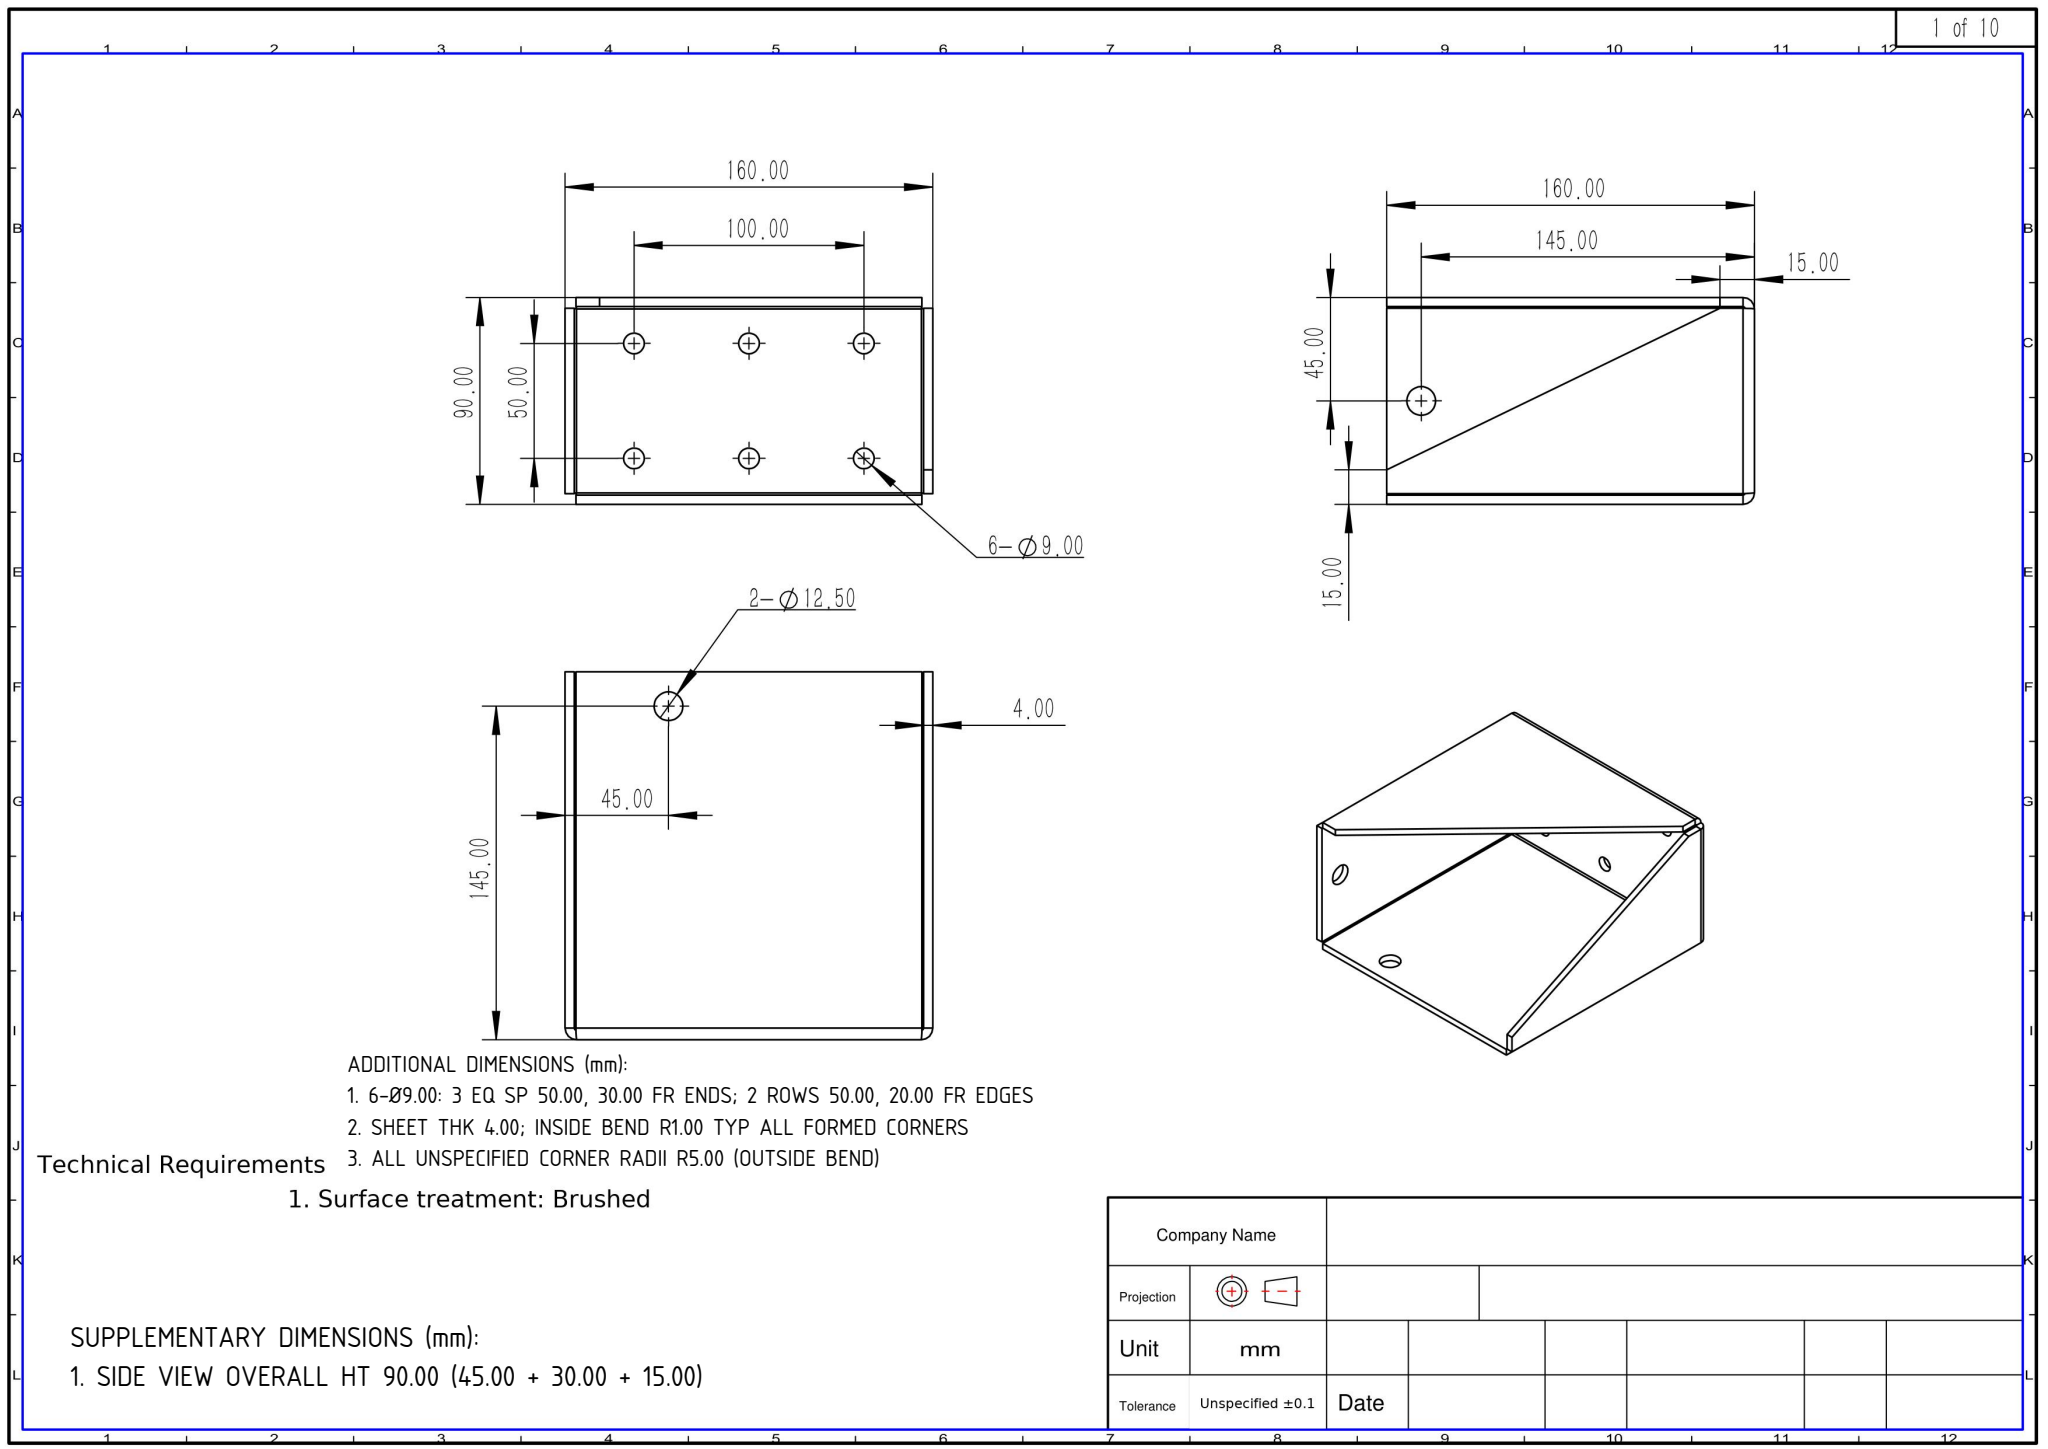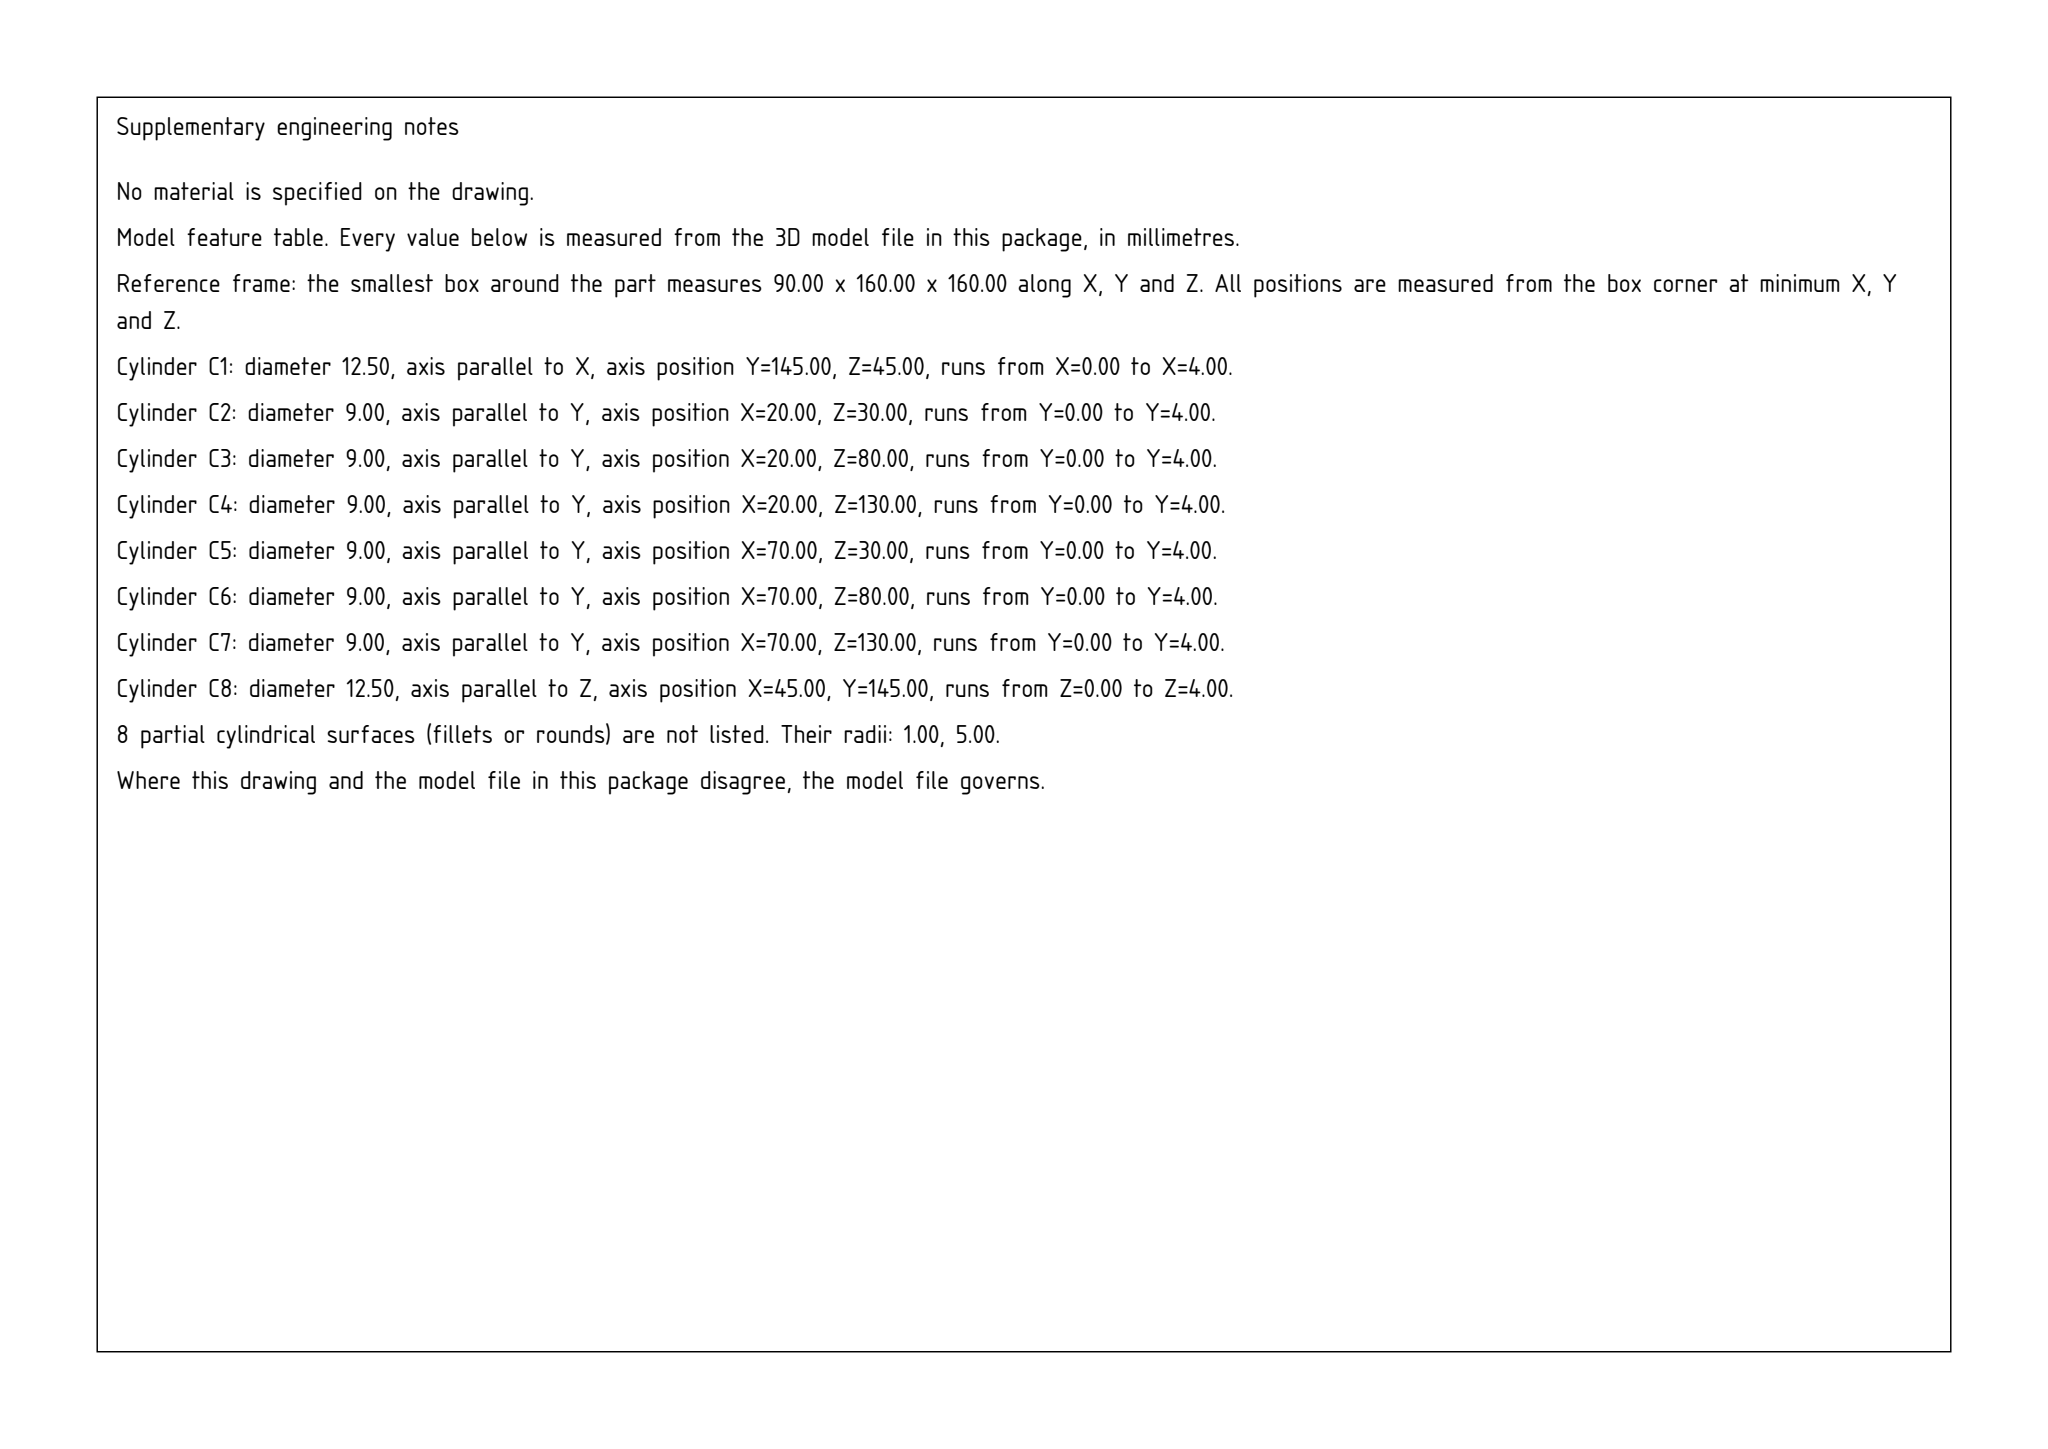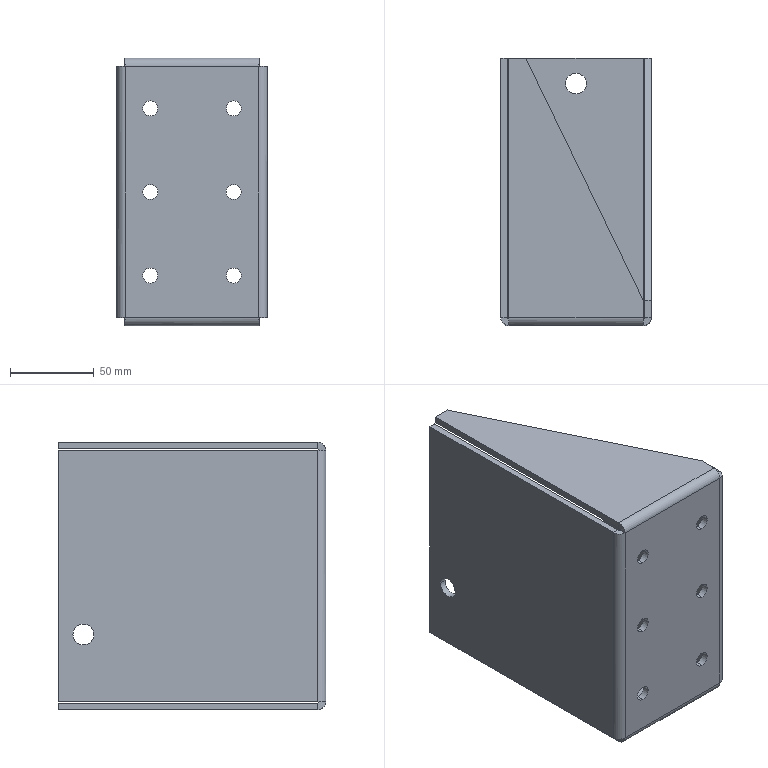Part | SolidWorks | mm | 1 solid | 56 faces | box 90 x 160 x 160 mm | volume 279767 mm3 | cylinder 24 | plane 24 | spline 8 | commonest cylinder face diameters 9 x12 12.5 x4 10 x4 2 x4